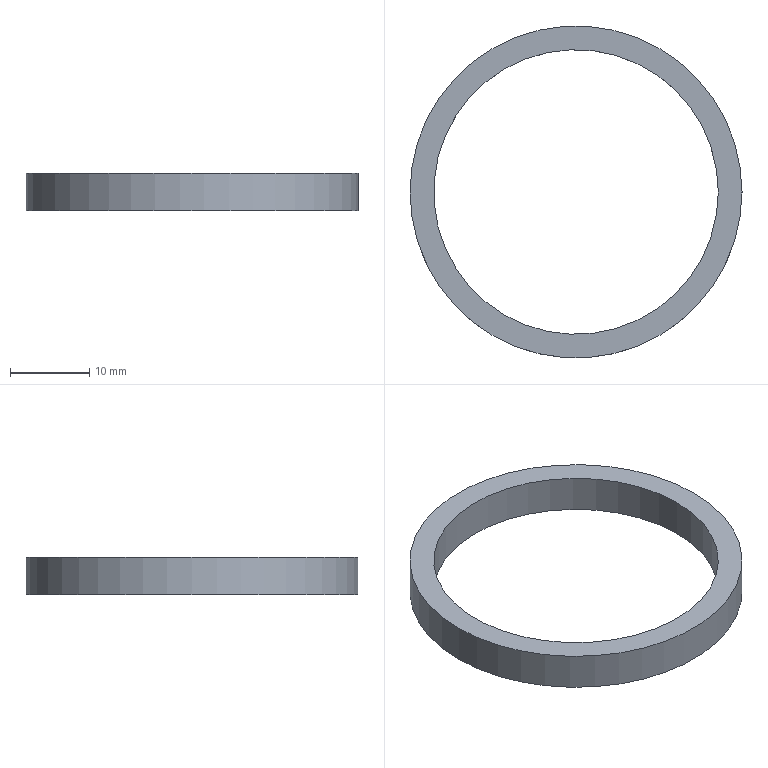Component | NX | O_RING | 1 solid | 4 faces | box 42 x 42 x 4.8 mm | volume 1764 mm3 | cylinder 2 | plane 2 | commonest cylinder face diameters 42 x1 36 x1
STEP:
#1=CARTESIAN_POINT('',(0.,0.,0.));
#2=DIRECTION('',(0.,0.,1.));
#3=DIRECTION('',(1.,0.,0.));
#4=AXIS2_PLACEMENT_3D('',#1,#2,#3);
#5=CARTESIAN_POINT('',(21.,-0.,105.7));
#6=VERTEX_POINT('',#5);
#7=CARTESIAN_POINT('',(0.,-0.,105.7));
#8=DIRECTION('',(0.,0.,1.));
#9=DIRECTION('',(1.,-0.,0.));
#10=AXIS2_PLACEMENT_3D('',#7,#8,#9);
#11=CIRCLE('',#10,21.);
#12=CARTESIAN_POINT('',(0.,-0.,105.7));
#13=DIRECTION('',(0.,0.,1.));
#14=DIRECTION('',(-1.,0.,0.));
#15=AXIS2_PLACEMENT_3D('',#12,#13,#14);
#16=CYLINDRICAL_SURFACE('',#15,21.);
#17=CARTESIAN_POINT('',(3.142,0.));
#18=DIRECTION('',(1.,0.));
#19=VECTOR('',#18,1.);
#20=LINE('',#17,#19);
#21=(GEOMETRIC_REPRESENTATION_CONTEXT(2)PARAMETRIC_REPRESENTATION_CONTEXT()REPRESENTATION_CONTEXT('',''));
#22=DEFINITIONAL_REPRESENTATION('',(#20),#21);
#23=PCURVE('',#16,#22);
#24=CARTESIAN_POINT('',(0.,-0.,105.7));
#25=DIRECTION('',(0.,0.,1.));
#26=DIRECTION('',(-1.,0.,0.));
#27=AXIS2_PLACEMENT_3D('',#24,#25,#26);
#28=PLANE('',#27);
#29=CARTESIAN_POINT('',(0.,0.));
#30=DIRECTION('',(-1.,0.));
#31=AXIS2_PLACEMENT_2D('',#29,#30);
#32=CIRCLE('',#31,21.);
#33=(GEOMETRIC_REPRESENTATION_CONTEXT(2)PARAMETRIC_REPRESENTATION_CONTEXT()REPRESENTATION_CONTEXT('',''));
#34=DEFINITIONAL_REPRESENTATION('',(#32),#33);
#35=PCURVE('',#28,#34);
#36=SURFACE_CURVE('',#11,(#23,#35),.PCURVE_S1.);
#37=EDGE_CURVE('',#6,#6,#36,.T.);
#38=ORIENTED_EDGE('',*,*,#37,.T.);
#39=CARTESIAN_POINT('',(21.,-0.,110.5));
#40=VERTEX_POINT('',#39);
#41=CARTESIAN_POINT('',(21.,-0.,105.7));
#42=CARTESIAN_POINT('',(21.,-0.,110.5));
#43=B_SPLINE_CURVE_WITH_KNOTS('',1,(#41,#42),.UNSPECIFIED.,.F.,.F.,(2,2),(0.,4.8),.PIECEWISE_BEZIER_KNOTS.);
#44=CARTESIAN_POINT('',(9.425,0.));
#45=DIRECTION('',(0.,1.));
#46=VECTOR('',#45,1.);
#47=LINE('',#44,#46);
#48=(GEOMETRIC_REPRESENTATION_CONTEXT(2)PARAMETRIC_REPRESENTATION_CONTEXT()REPRESENTATION_CONTEXT('',''));
#49=DEFINITIONAL_REPRESENTATION('',(#47),#48);
#50=PCURVE('',#16,#49);
#51=CARTESIAN_POINT('',(3.142,0.));
#52=DIRECTION('',(0.,1.));
#53=VECTOR('',#52,1.);
#54=LINE('',#51,#53);
#55=(GEOMETRIC_REPRESENTATION_CONTEXT(2)PARAMETRIC_REPRESENTATION_CONTEXT()REPRESENTATION_CONTEXT('',''));
#56=DEFINITIONAL_REPRESENTATION('',(#54),#55);
#57=PCURVE('',#16,#56);
#58=SEAM_CURVE('',#43,(#50,#57),.PCURVE_S1.);
#59=EDGE_CURVE('',#6,#40,#58,.T.);
#60=ORIENTED_EDGE('',*,*,#59,.T.);
#61=CARTESIAN_POINT('',(0.,-0.,110.5));
#62=DIRECTION('',(0.,0.,1.));
#63=DIRECTION('',(1.,-0.,0.));
#64=AXIS2_PLACEMENT_3D('',#61,#62,#63);
#65=CIRCLE('',#64,21.);
#66=CARTESIAN_POINT('',(3.142,4.8));
#67=DIRECTION('',(1.,0.));
#68=VECTOR('',#67,1.);
#69=LINE('',#66,#68);
#70=(GEOMETRIC_REPRESENTATION_CONTEXT(2)PARAMETRIC_REPRESENTATION_CONTEXT()REPRESENTATION_CONTEXT('',''));
#71=DEFINITIONAL_REPRESENTATION('',(#69),#70);
#72=PCURVE('',#16,#71);
#73=CARTESIAN_POINT('',(0.,-0.,110.5));
#74=DIRECTION('',(0.,0.,1.));
#75=DIRECTION('',(-1.,0.,0.));
#76=AXIS2_PLACEMENT_3D('',#73,#74,#75);
#77=PLANE('',#76);
#78=CARTESIAN_POINT('',(0.,0.));
#79=DIRECTION('',(-1.,0.));
#80=AXIS2_PLACEMENT_2D('',#78,#79);
#81=CIRCLE('',#80,21.);
#82=(GEOMETRIC_REPRESENTATION_CONTEXT(2)PARAMETRIC_REPRESENTATION_CONTEXT()REPRESENTATION_CONTEXT('',''));
#83=DEFINITIONAL_REPRESENTATION('',(#81),#82);
#84=PCURVE('',#77,#83);
#85=SURFACE_CURVE('',#65,(#72,#84),.PCURVE_S1.);
#86=EDGE_CURVE('',#40,#40,#85,.T.);
#87=ORIENTED_EDGE('',*,*,#86,.F.);
#88=ORIENTED_EDGE('',*,*,#59,.F.);
#89=EDGE_LOOP('',(#38,#60,#87,#88));
#90=FACE_BOUND('',#89,.T.);
#91=ADVANCED_FACE('',(#90),#16,.T.);
#92=CARTESIAN_POINT('',(18.,-0.,105.7));
#93=VERTEX_POINT('',#92);
#94=CARTESIAN_POINT('',(0.,-0.,105.7));
#95=DIRECTION('',(0.,0.,1.));
#96=DIRECTION('',(1.,-0.,0.));
#97=AXIS2_PLACEMENT_3D('',#94,#95,#96);
#98=CIRCLE('',#97,18.);
#99=CARTESIAN_POINT('',(0.,-0.,105.7));
#100=DIRECTION('',(0.,0.,1.));
#101=DIRECTION('',(-1.,0.,0.));
#102=AXIS2_PLACEMENT_3D('',#99,#100,#101);
#103=CYLINDRICAL_SURFACE('',#102,18.);
#104=CARTESIAN_POINT('',(3.142,0.));
#105=DIRECTION('',(1.,0.));
#106=VECTOR('',#105,1.);
#107=LINE('',#104,#106);
#108=(GEOMETRIC_REPRESENTATION_CONTEXT(2)PARAMETRIC_REPRESENTATION_CONTEXT()REPRESENTATION_CONTEXT('',''));
#109=DEFINITIONAL_REPRESENTATION('',(#107),#108);
#110=PCURVE('',#103,#109);
#111=CARTESIAN_POINT('',(0.,0.));
#112=DIRECTION('',(-1.,0.));
#113=AXIS2_PLACEMENT_2D('',#111,#112);
#114=CIRCLE('',#113,18.);
#115=(GEOMETRIC_REPRESENTATION_CONTEXT(2)PARAMETRIC_REPRESENTATION_CONTEXT()REPRESENTATION_CONTEXT('',''));
#116=DEFINITIONAL_REPRESENTATION('',(#114),#115);
#117=PCURVE('',#28,#116);
#118=SURFACE_CURVE('',#98,(#110,#117),.PCURVE_S1.);
#119=EDGE_CURVE('',#93,#93,#118,.T.);
#120=ORIENTED_EDGE('',*,*,#119,.T.);
#121=CARTESIAN_POINT('',(18.,-0.,110.5));
#122=VERTEX_POINT('',#121);
#123=CARTESIAN_POINT('',(18.,-0.,105.7));
#124=CARTESIAN_POINT('',(18.,-0.,110.5));
#125=B_SPLINE_CURVE_WITH_KNOTS('',1,(#123,#124),.UNSPECIFIED.,.F.,.F.,(2,2),(0.,4.8),.PIECEWISE_BEZIER_KNOTS.);
#126=CARTESIAN_POINT('',(9.425,0.));
#127=DIRECTION('',(0.,1.));
#128=VECTOR('',#127,1.);
#129=LINE('',#126,#128);
#130=(GEOMETRIC_REPRESENTATION_CONTEXT(2)PARAMETRIC_REPRESENTATION_CONTEXT()REPRESENTATION_CONTEXT('',''));
#131=DEFINITIONAL_REPRESENTATION('',(#129),#130);
#132=PCURVE('',#103,#131);
#133=CARTESIAN_POINT('',(3.142,0.));
#134=DIRECTION('',(0.,1.));
#135=VECTOR('',#134,1.);
#136=LINE('',#133,#135);
#137=(GEOMETRIC_REPRESENTATION_CONTEXT(2)PARAMETRIC_REPRESENTATION_CONTEXT()REPRESENTATION_CONTEXT('',''));
#138=DEFINITIONAL_REPRESENTATION('',(#136),#137);
#139=PCURVE('',#103,#138);
#140=SEAM_CURVE('',#125,(#132,#139),.PCURVE_S1.);
#141=EDGE_CURVE('',#93,#122,#140,.T.);
#142=ORIENTED_EDGE('',*,*,#141,.T.);
#143=CARTESIAN_POINT('',(0.,-0.,110.5));
#144=DIRECTION('',(0.,0.,1.));
#145=DIRECTION('',(1.,-0.,0.));
#146=AXIS2_PLACEMENT_3D('',#143,#144,#145);
#147=CIRCLE('',#146,18.);
#148=CARTESIAN_POINT('',(3.142,4.8));
#149=DIRECTION('',(1.,0.));
#150=VECTOR('',#149,1.);
#151=LINE('',#148,#150);
#152=(GEOMETRIC_REPRESENTATION_CONTEXT(2)PARAMETRIC_REPRESENTATION_CONTEXT()REPRESENTATION_CONTEXT('',''));
#153=DEFINITIONAL_REPRESENTATION('',(#151),#152);
#154=PCURVE('',#103,#153);
#155=CARTESIAN_POINT('',(0.,0.));
#156=DIRECTION('',(-1.,0.));
#157=AXIS2_PLACEMENT_2D('',#155,#156);
#158=CIRCLE('',#157,18.);
#159=(GEOMETRIC_REPRESENTATION_CONTEXT(2)PARAMETRIC_REPRESENTATION_CONTEXT()REPRESENTATION_CONTEXT('',''));
#160=DEFINITIONAL_REPRESENTATION('',(#158),#159);
#161=PCURVE('',#77,#160);
#162=SURFACE_CURVE('',#147,(#154,#161),.PCURVE_S1.);
#163=EDGE_CURVE('',#122,#122,#162,.T.);
#164=ORIENTED_EDGE('',*,*,#163,.F.);
#165=ORIENTED_EDGE('',*,*,#141,.F.);
#166=EDGE_LOOP('',(#120,#142,#164,#165));
#167=FACE_BOUND('',#166,.F.);
#168=ADVANCED_FACE('',(#167),#103,.F.);
#169=ORIENTED_EDGE('',*,*,#37,.F.);
#170=EDGE_LOOP('',(#169));
#171=FACE_BOUND('',#170,.T.);
#172=ORIENTED_EDGE('',*,*,#119,.T.);
#173=EDGE_LOOP('',(#172));
#174=FACE_BOUND('',#173,.T.);
#175=ADVANCED_FACE('',(#171,#174),#28,.F.);
#176=ORIENTED_EDGE('',*,*,#86,.T.);
#177=EDGE_LOOP('',(#176));
#178=FACE_BOUND('',#177,.T.);
#179=ORIENTED_EDGE('',*,*,#163,.F.);
#180=EDGE_LOOP('',(#179));
#181=FACE_BOUND('',#180,.T.);
#182=ADVANCED_FACE('',(#178,#181),#77,.T.);
#183=CLOSED_SHELL('',(#91,#168,#175,#182));
#184=MANIFOLD_SOLID_BREP('',#183);
#185=(LENGTH_UNIT()NAMED_UNIT(*)SI_UNIT(.MILLI.,.METRE.));
#186=UNCERTAINTY_MEASURE_WITH_UNIT(LENGTH_MEASURE(0.00001),#185,'','');
#187=(NAMED_UNIT(*)PLANE_ANGLE_UNIT()SI_UNIT($,.RADIAN.));
#188=(NAMED_UNIT(*)SI_UNIT($,.STERADIAN.)SOLID_ANGLE_UNIT());
#189=(GEOMETRIC_REPRESENTATION_CONTEXT(3)GLOBAL_UNCERTAINTY_ASSIGNED_CONTEXT((#186))GLOBAL_UNIT_ASSIGNED_CONTEXT((#185,#187,#188))REPRESENTATION_CONTEXT('',''));
#190=ADVANCED_BREP_SHAPE_REPRESENTATION('',(#4,#184),#189);